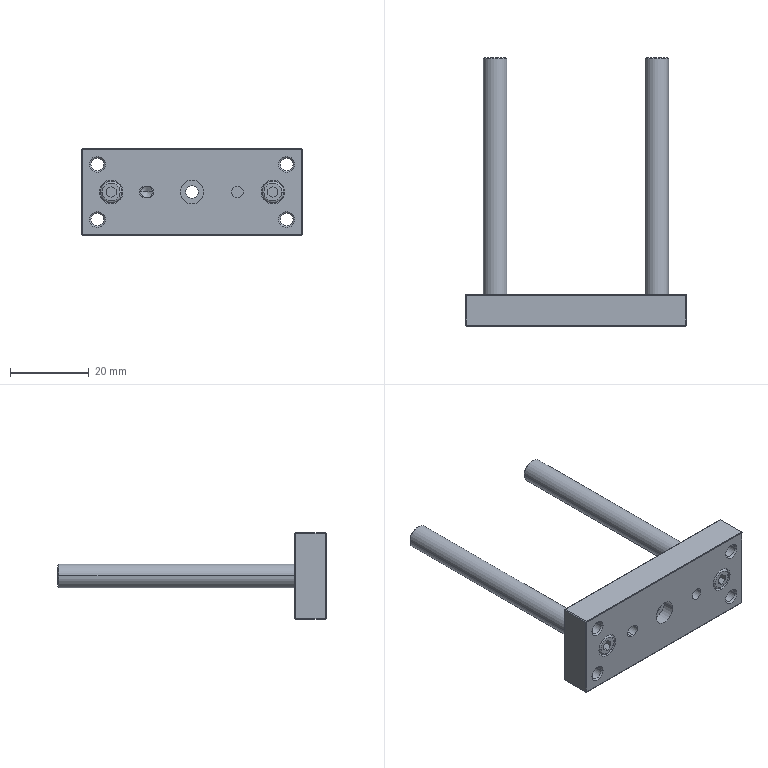Component | SolidWorks | TC_L_12x30_S_0-1_TC_L_12x30_30fp-1 | 1 solid | 101 faces | box 56 x 68 x 22 mm | volume 12698 mm3 | plane 44 | cylinder 31 | cone 22 | torus 4 | commonest cylinder face diameters 6 x10 3.242 x8 3 x7 5.5 x4 3.2 x2
build123d program:
from build123d import *

# Parameters (mm, degrees)
BOSS_EXTRUDE1_DEPTH     = 8
CUT_EXTRUDE1_DEPTH      = 26
CUT_EXTRUDE1_DEPTH_BACK = 26
SKETCH2_W               = 24
SKETCH2_H               = 72
CUT_EXTRUDE2_DEPTH      = 56
CUT_EXTRUDE2_DEPTH_BACK = 56
SKETCH3_W               = 24
SKETCH3_H               = 38
CUT_EXTRUDE3_DEPTH      = 2
CUT_EXTRUDE4_DEPTH      = 2
LPATTERN1_COUNT         = 2
LPATTERN1_PITCH         = 48
LPATTERN1_COUNT_DIR2    = 2
LPATTERN1_PITCH_DIR2    = 14
SKETCH12_W              = 6
SKETCH12_H              = 1.5
CUT_EXTRUDE5_DEPTH      = 3


with BuildPart() as part:
    # Sketch1 → Boss-Extrude1 (new body)
    with BuildSketch(Plane(origin=(0, 0, 0), x_dir=(0, 0, -1), z_dir=(1, 0, 0))):
        Polygon((-28, 10.8), (-28, -10.8), (-27.8, -11), (27.8, -11), (28, -10.8), (28, 10.8), (27.8, 11), (-27.8, 11), align=None)
    extrude(amount=BOSS_EXTRUDE1_DEPTH)

    # Sketch2 → Cut-Extrude1 (cut, two sides: drawn at the far end of the back side and taken through both)
    with BuildSketch(Plane(origin=(0, 0, 0), x_dir=(1, 0, 0), z_dir=(0, 1, 0)).offset(-CUT_EXTRUDE1_DEPTH_BACK)):
        with Locations((4, 0)):
            Rectangle(SKETCH2_W, SKETCH2_H)
        Polygon((0, 27.8), (0, -27.8), (0.2, -28), (7.8, -28), (8, -27.8), (8, 27.8), (7.8, 28), (0.2, 28), align=None, mode=Mode.SUBTRACT)
    extrude(amount=CUT_EXTRUDE1_DEPTH + CUT_EXTRUDE1_DEPTH_BACK, mode=Mode.SUBTRACT)

    # Sketch3 → Cut-Extrude2 (cut, two sides: drawn at the far end of the back side and taken through both)
    with BuildSketch(Plane.XY.offset(-CUT_EXTRUDE2_DEPTH_BACK)):
        with Locations((4, 0)):
            Rectangle(SKETCH3_W, SKETCH3_H)
        Polygon((0, 10.8), (0, -10.8), (0.2, -11), (7.8, -11), (8, -10.8), (8, 10.8), (7.8, 11), (0.2, 11), align=None, mode=Mode.SUBTRACT)
    extrude(amount=CUT_EXTRUDE2_DEPTH + CUT_EXTRUDE2_DEPTH_BACK, mode=Mode.SUBTRACT)

    # Sketch4 → Cut-Revolve1 (revolve, cut)
    with BuildSketch(Plane.XY.offset(20.5), mode=Mode.PRIVATE) as cut_revolve1_sk:
        with BuildLine():
            Line((0, 3), (0, 2.25))
            ThreePointArc((0, 2.25), (0.1464, 2.604), (0.5, 2.75))
            Line((0.5, 2.75), (3.5, 2.75))
            Line((3.5, 2.75), (3.5, 3))
            Line((3.5, 3), (0, 3))
        make_face()
    revolve(cut_revolve1_sk.sketch.rotate(Axis((3.5, 0, 20.5), (-1, 0, 0)), 270), axis=Axis((3.5, 0, 20.5), (-1, 0, 0)), mode=Mode.SUBTRACT)

    # Sketch5 → Cut-Revolve2 (revolve, cut)
    with BuildSketch(Plane.XY.offset(-20.5), mode=Mode.PRIVATE) as cut_revolve2_sk:
        with BuildLine():
            Line((0, 3), (0, 2.25))
            ThreePointArc((0, 2.25), (0.1464, 2.604), (0.5, 2.75))
            Line((0.5, 2.75), (3.5, 2.75))
            Line((3.5, 2.75), (3.5, 3))
            Line((3.5, 3), (0, 3))
        make_face()
    revolve(cut_revolve2_sk.sketch.rotate(Axis((3.5, 0, -20.5), (-1, 0, 0)), 270), axis=Axis((3.5, 0, -20.5), (-1, 0, 0)), mode=Mode.SUBTRACT)

    # Sketch6 → Cut-Extrude3 (cut)
    with BuildSketch(Plane(origin=(0, 0, 0), x_dir=(0, 0, -1), z_dir=(1, 0, 0))):
        Polygon((-21.75, 0.7217), (-21.75, -0.7217), (-20.5, -1.443), (-19.25, -0.7217), (-19.25, 0.7217), (-20.5, 1.443), align=None)
    extrude(amount=CUT_EXTRUDE3_DEPTH, mode=Mode.SUBTRACT)

    # Sketch7 → Cut-Extrude4 (cut)
    with BuildSketch(Plane(origin=(0, 0, 0), x_dir=(0, 0, -1), z_dir=(1, 0, 0))):
        Polygon((19.25, 0.7217), (19.25, -0.7217), (20.5, -1.443), (21.75, -0.7217), (21.75, 0.7217), (20.5, 1.443), align=None)
    extrude(amount=CUT_EXTRUDE4_DEPTH, mode=Mode.SUBTRACT)

    # Sketch8 → Revolve1 (revolve)
    with BuildSketch(Plane.XY.offset(20.5), mode=Mode.PRIVATE) as revolve1_sk:
        Polygon((8, 0), (8, 3), (67.75, 3), (68, 2.75), (68, 0), align=None)
    revolve(revolve1_sk.sketch.rotate(Axis((68, 0, 20.5), (-1, 0, 0)), 270), axis=Axis((68, 0, 20.5), (-1, 0, 0)))

    # Sketch9 → Revolve2 (revolve)
    with BuildSketch(Plane.XY.offset(-20.5), mode=Mode.PRIVATE) as revolve2_sk:
        Polygon((8, 0), (8, 3), (67.75, 3), (68, 2.75), (68, 0), align=None)
    revolve(revolve2_sk.sketch.rotate(Axis((68, 0, -20.5), (-1, 0, 0)), 270), axis=Axis((68, 0, -20.5), (-1, 0, 0)))

    # Sketch10 → Cut-Revolve3 (revolve, cut)
    with BuildSketch(Plane.XY.offset(24), mode=Mode.PRIVATE) as cut_revolve3_sk:
        Polygon((0, -7), (0, -5), (0.379, -5.379), (7.621, -5.379), (8, -5), (8, -7), align=None)
    cut_revolve3 = revolve(cut_revolve3_sk.sketch.rotate(Axis((8, -7, 24), (-1, 0, 0)), 270), axis=Axis((8, -7, 24), (-1, 0, 0)), mode=Mode.SUBTRACT)

    # LPattern1: Cut-Revolve3 2 × 2
    with Locations(*[(0, j * LPATTERN1_PITCH_DIR2, -i * LPATTERN1_PITCH) for i in range(LPATTERN1_COUNT) for j in range(LPATTERN1_COUNT_DIR2) if (i, j) != (0, 0)]):
        add(cut_revolve3, mode=Mode.SUBTRACT)

    # Sketch12 → Cut-Revolve4 (revolve, cut)
    with BuildSketch(Plane.XY.offset(11.5), mode=Mode.PRIVATE) as cut_revolve4_sk:
        with Locations((3, 0.75)):
            Rectangle(SKETCH12_W, SKETCH12_H)
    revolve(cut_revolve4_sk.sketch.rotate(Axis((6, 0, 11.5), (-1, 0, 0)), 270), axis=Axis((6, 0, 11.5), (-1, 0, 0)), mode=Mode.SUBTRACT)

    # Sketch13 → Cut-Revolve5 (revolve, cut)
    with BuildSketch(Plane.XY.offset(-11.5), mode=Mode.PRIVATE) as cut_revolve5_sk:
        Polygon((0, 0), (0, 1.5), (6, 1.5), (6.866, 0), align=None)
    revolve(cut_revolve5_sk.sketch.rotate(Axis((6.866, 0, -11.5), (-1, 0, 0)), 270), axis=Axis((6.866, 0, -11.5), (-1, 0, 0)), mode=Mode.SUBTRACT)

    # Sketch14 → Cut-Extrude5 (cut)
    with BuildSketch(Plane(origin=(0, 0, 0), x_dir=(0, 0, -1), z_dir=(1, 0, 0))):
        with BuildLine():
            Line((11.2, -1.5), (11.8, -1.5))
            ThreePointArc((11.8, -1.5), (13.3, 0), (11.8, 1.5))
            Line((11.8, 1.5), (11.2, 1.5))
            ThreePointArc((11.2, 1.5), (9.7, 0), (11.2, -1.5))
        make_face()
    extrude(amount=CUT_EXTRUDE5_DEPTH, mode=Mode.SUBTRACT)

    # Sketch15 → Cut-Revolve6 (revolve, cut)
    with BuildSketch(Plane.XY, mode=Mode.PRIVATE) as cut_revolve6_sk:
        Polygon((0, 0), (0, 3), (3, 3), (3, 1.6), (8, 1.6), (8, 0), align=None)
    revolve(cut_revolve6_sk.sketch.rotate(Axis((8, 0, 0), (-1, 0, 0)), 270), axis=Axis((8, 0, 0), (-1, 0, 0)), mode=Mode.SUBTRACT)


solid = part.part

# Placed as in the assembly
solid = solid.moved(Location((-42, 161.3, 57), (90, 90, 0)))